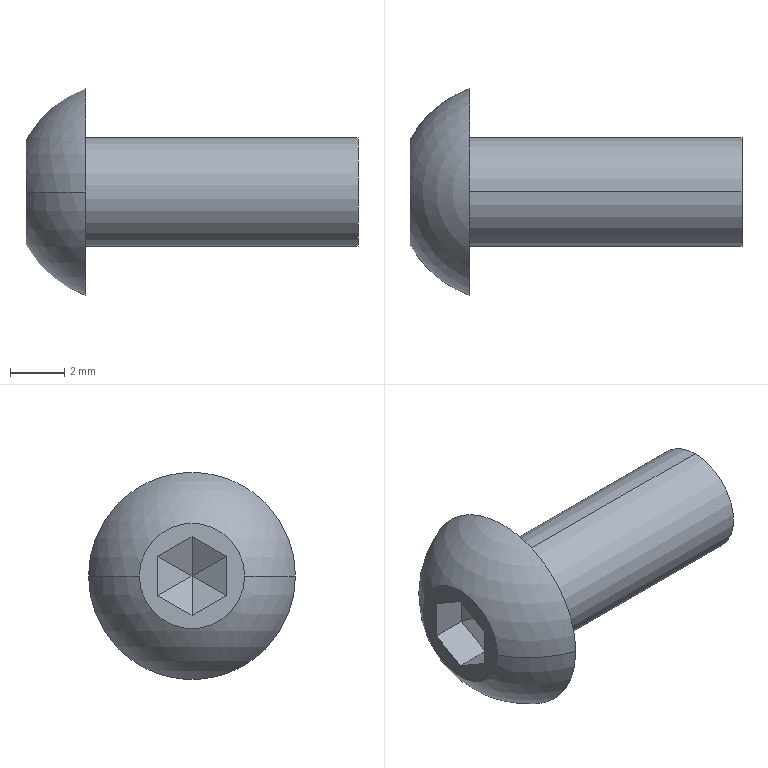Component | SolidWorks | hexagon socket button head screws gb-6 | 1 solid | 19 faces | volume 186 mm3 | plane 15 | sphere 2 | cylinder 2 | commonest cylinder face diameters 4 x2